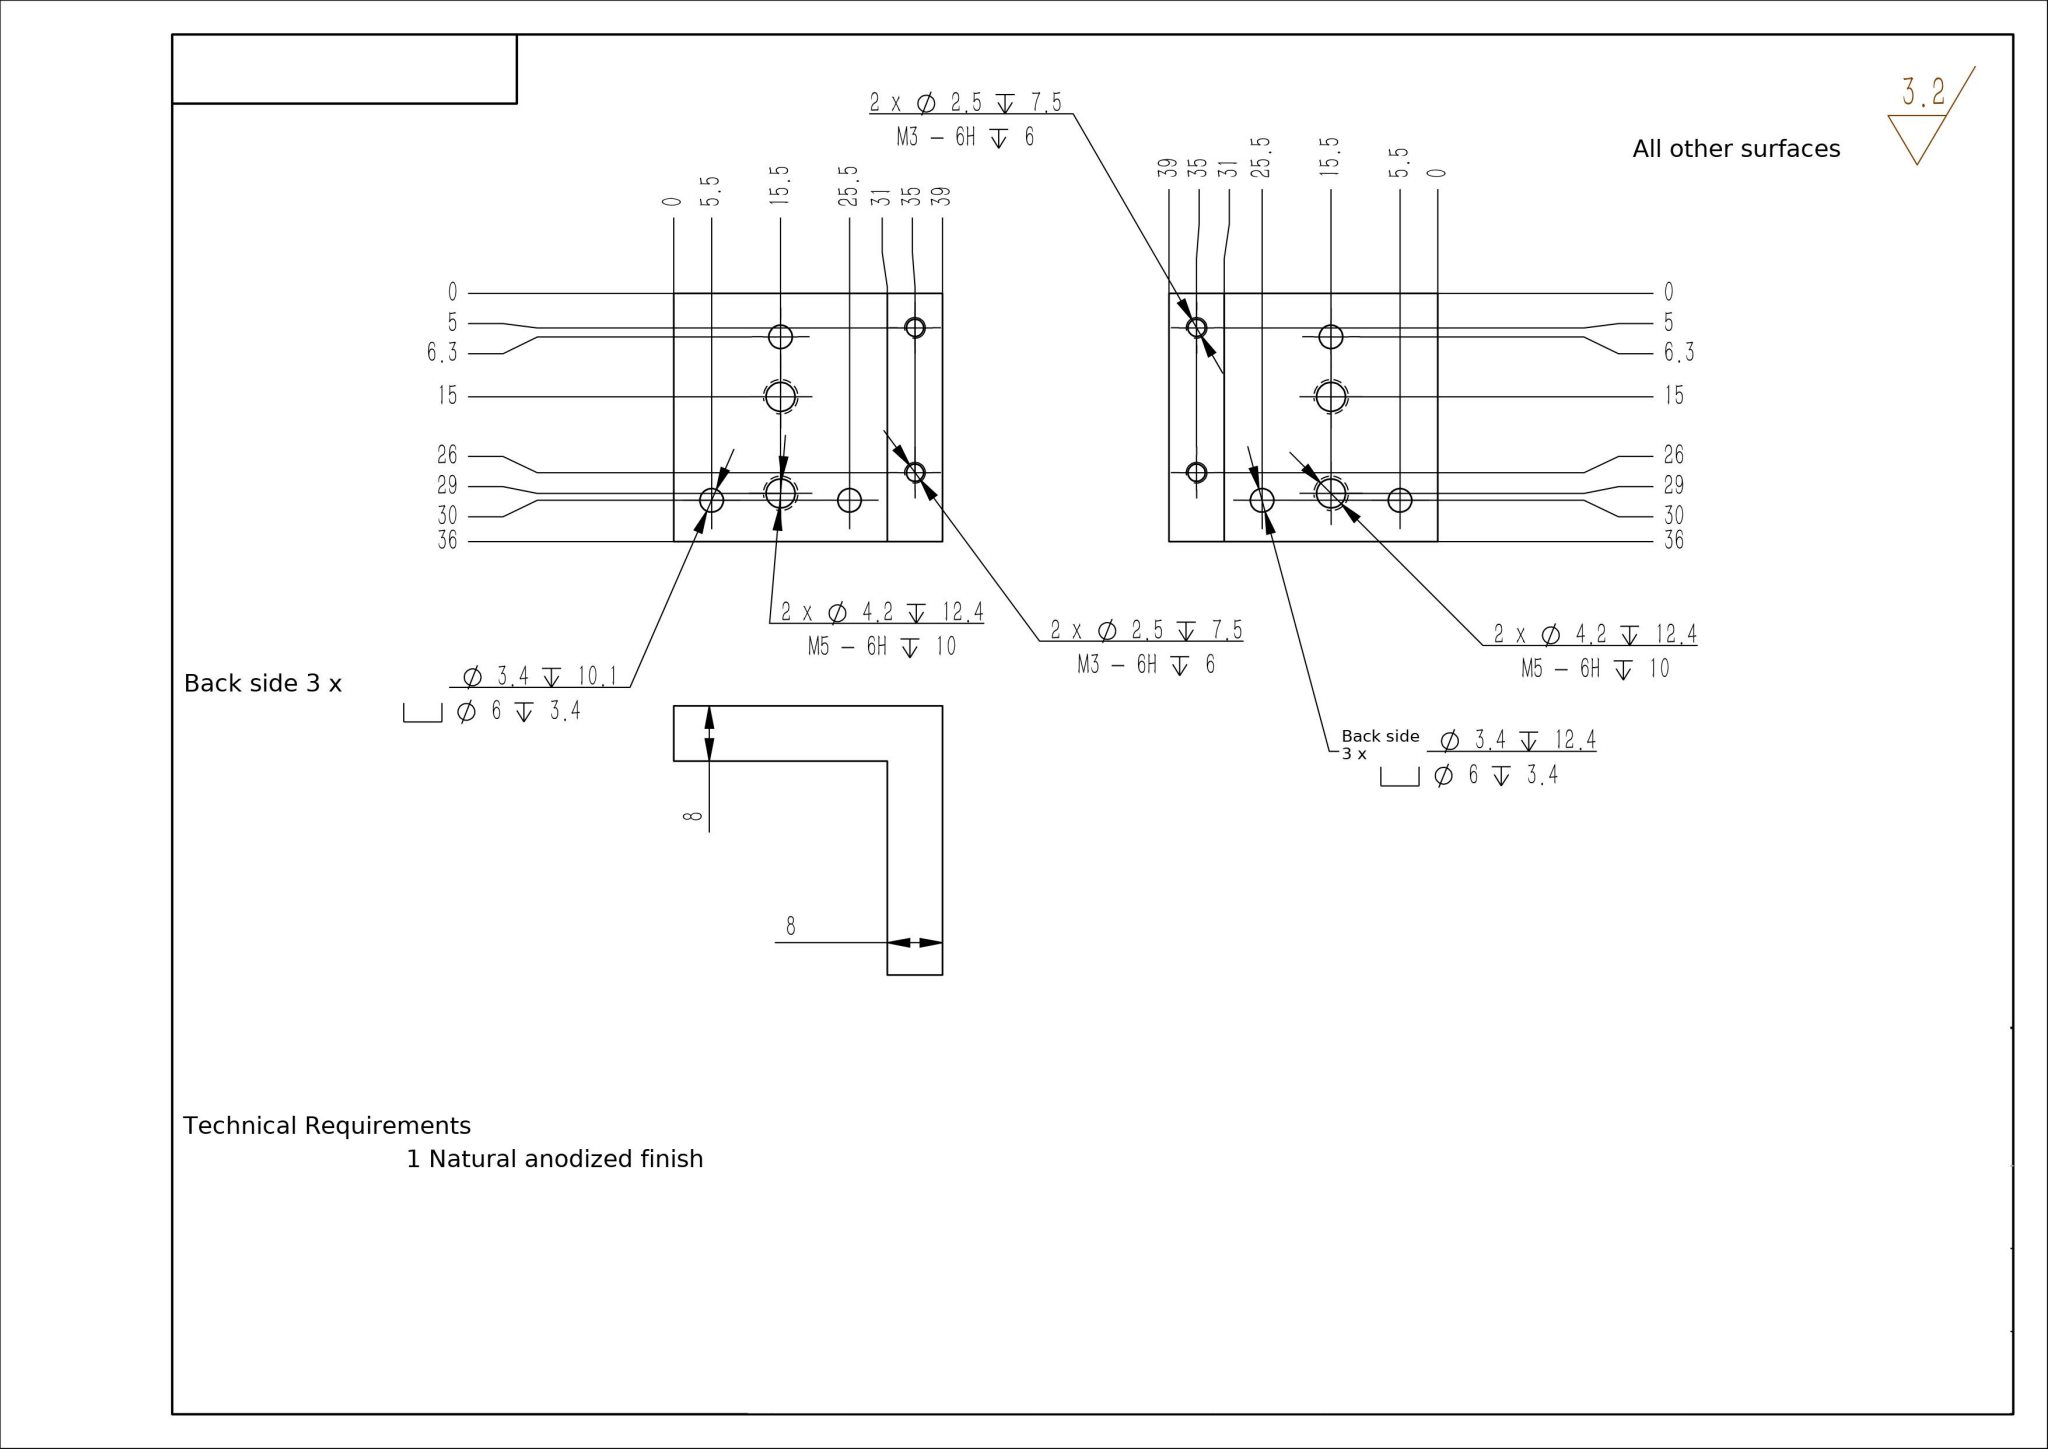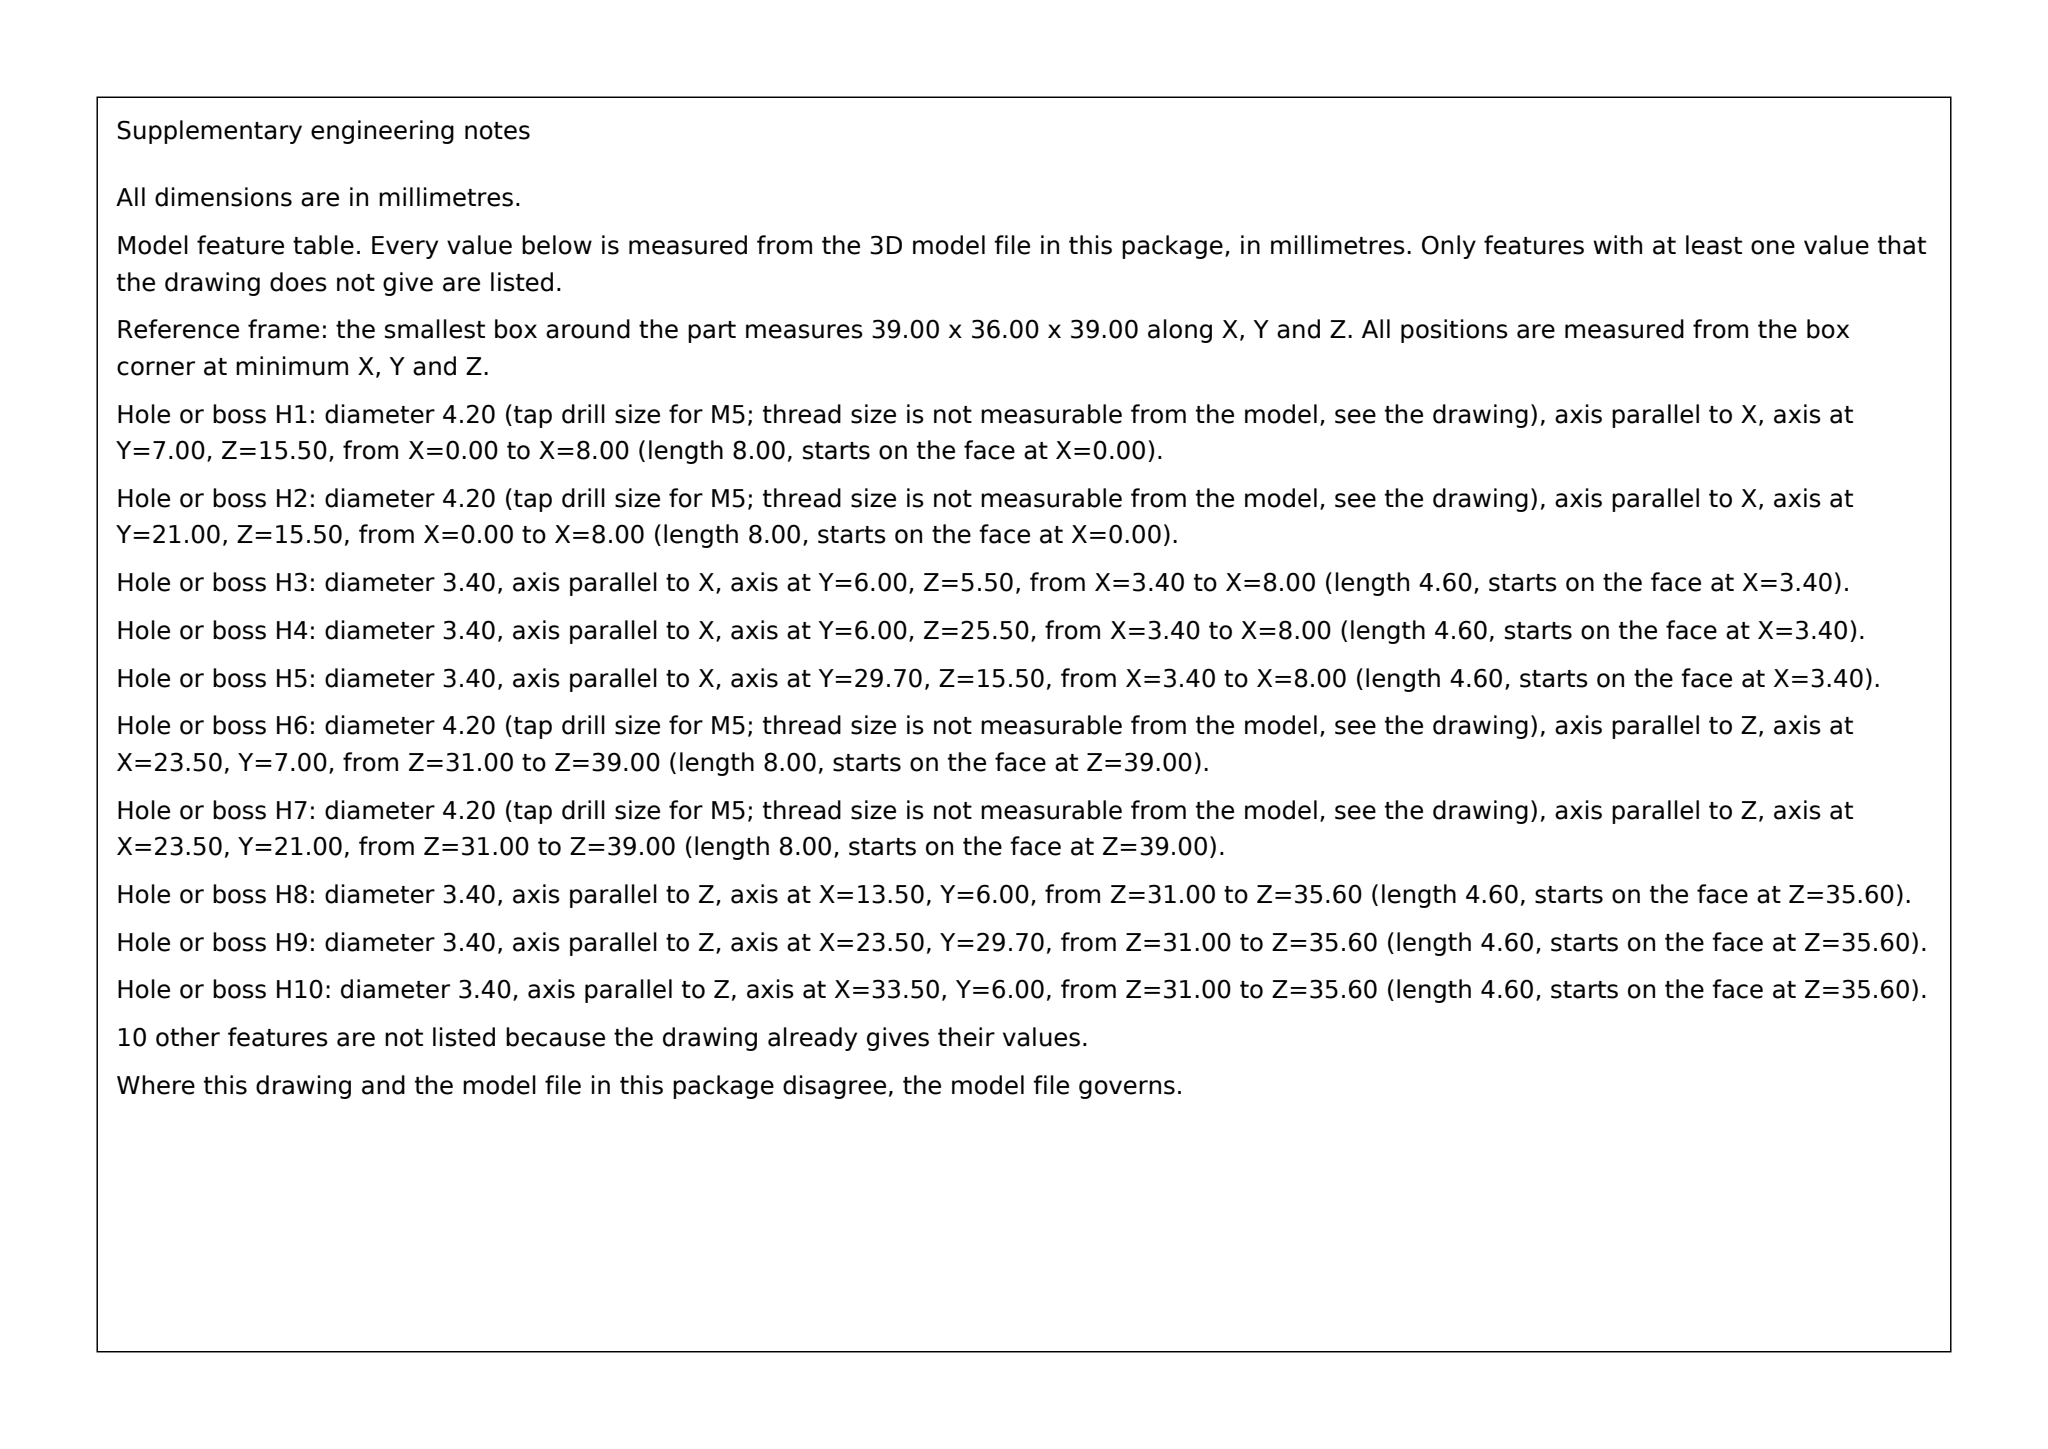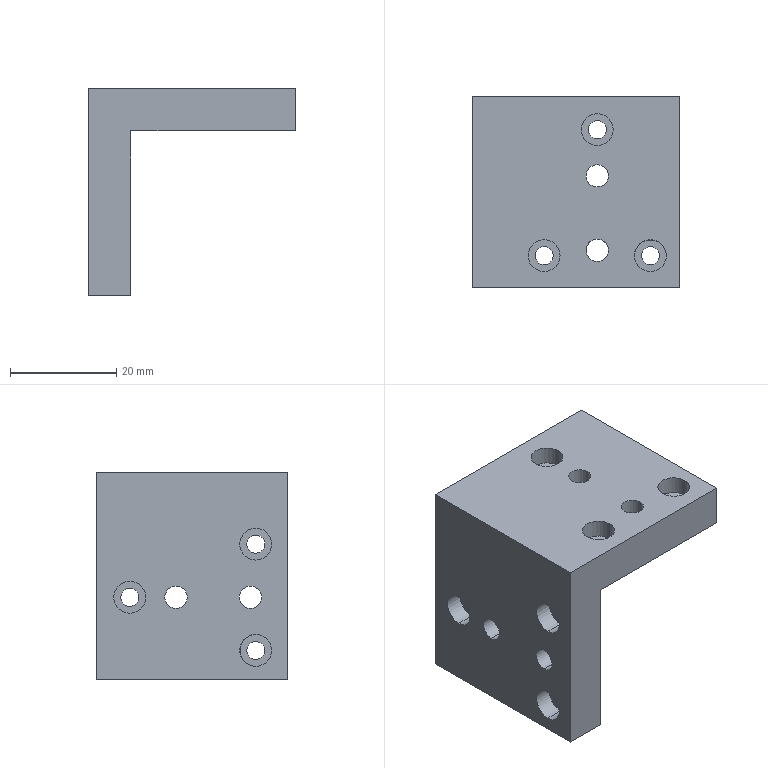Part | SolidWorks | mm | 1 solid | 62 faces | box 39 x 36 x 39 mm | volume 18737 mm3 | cylinder 40 | plane 14 | cone 8 | commonest cylinder face diameters 6 x12 3.4 x12 2.5 x8 4.2 x8
build123d program:
from build123d import *

# Parameters (mm, degrees)
BOSS_EXTRUDE1_DEPTH                               = 36
HOLE_SIZE_ACCORDING_TO_HEXAGON_SOCKET_D           = 3.4
HOLE_SIZE_ACCORDING_TO_HEXAGON_SOCKET_DEPTH       = 10.1
HOLE_SIZE_ACCORDING_TO_HEXAGON_SOCKET_CBORE_D     = 6
HOLE_SIZE_ACCORDING_TO_HEXAGON_SOCKET_CBORE_DEPTH = 3.4
HOLE_SIZE_ACCORDING_TO_HEXAGON_SOCKET_TIP         = 1.021
M5_TAPPED_HOLE1_D                                 = 4.2
M5_TAPPED_HOLE1_DEPTH                             = 12.4
M5_TAPPED_HOLE1_TIP                               = 1.262
HOLE_SIZE_ACCORDING_TO_HEXAGON_SO_2_D             = 3.4
HOLE_SIZE_ACCORDING_TO_HEXAGON_SO_2_DEPTH         = 12.4
HOLE_SIZE_ACCORDING_TO_HEXAGON_SO_2_CBORE_D       = 6
HOLE_SIZE_ACCORDING_TO_HEXAGON_SO_2_CBORE_DEPTH   = 3.4
HOLE_SIZE_ACCORDING_TO_HEXAGON_SO_2_TIP           = 1.021
M5_TAPPED_HOLE2_D                                 = 4.2
M5_TAPPED_HOLE2_DEPTH                             = 12.4
M5_TAPPED_HOLE2_TIP                               = 1.262
M3_TAPPED_HOLE1_D                                 = 2.5
M3_TAPPED_HOLE1_DEPTH                             = 7.5
M3_TAPPED_HOLE1_TIP                               = 0.7511
M3_TAPPED_HOLE2_D                                 = 2.5
M3_TAPPED_HOLE2_DEPTH                             = 7.5
M3_TAPPED_HOLE2_TIP                               = 0.7511


with BuildPart() as part:
    # Sketch1 → Boss-Extrude1 (new body)
    with BuildSketch(Plane(origin=(0, 0, 0), x_dir=(1, 0, 0), z_dir=(0, 1, 0))):
        Polygon((-16.522, 24.826), (-16.522, -14.174), (22.478, -14.174), (22.478, -6.174), (-8.522, -6.174), (-8.522, 24.826), align=None)
    extrude(amount=BOSS_EXTRUDE1_DEPTH)

    # Hole Size _ according to_ Hexagon Socket
    with Locations(Plane.XY.offset(14.174)):
        with Locations((6.978, 29.7), (-3.022, 6), (16.978, 6)):
            CounterBoreHole(HOLE_SIZE_ACCORDING_TO_HEXAGON_SOCKET_D / 2, HOLE_SIZE_ACCORDING_TO_HEXAGON_SOCKET_CBORE_D / 2, HOLE_SIZE_ACCORDING_TO_HEXAGON_SOCKET_CBORE_DEPTH, depth=HOLE_SIZE_ACCORDING_TO_HEXAGON_SOCKET_DEPTH)
            with Locations((0, 0, -(HOLE_SIZE_ACCORDING_TO_HEXAGON_SOCKET_DEPTH + HOLE_SIZE_ACCORDING_TO_HEXAGON_SOCKET_TIP / 2))):  # 118° drill point
                Cone(0, HOLE_SIZE_ACCORDING_TO_HEXAGON_SOCKET_D / 2, HOLE_SIZE_ACCORDING_TO_HEXAGON_SOCKET_TIP, mode=Mode.SUBTRACT)

    # M5 Tapped Hole1
    with Locations(Plane.XY.offset(14.174)):
        with Locations((6.977, 21), (6.977, 7)):
            Hole(M5_TAPPED_HOLE1_D / 2, depth=M5_TAPPED_HOLE1_DEPTH)
            with Locations((0, 0, -(M5_TAPPED_HOLE1_DEPTH + M5_TAPPED_HOLE1_TIP / 2))):  # 118° drill point
                Cone(0, M5_TAPPED_HOLE1_D / 2, M5_TAPPED_HOLE1_TIP, mode=Mode.SUBTRACT)

    # Hole Size _ according to_ Hexagon So 2
    with Locations(Plane.ZY.offset(16.522)):
        with Locations((-9.326, 29.7), (-19.326, 6), (0.6739, 6)):
            CounterBoreHole(HOLE_SIZE_ACCORDING_TO_HEXAGON_SO_2_D / 2, HOLE_SIZE_ACCORDING_TO_HEXAGON_SO_2_CBORE_D / 2, HOLE_SIZE_ACCORDING_TO_HEXAGON_SO_2_CBORE_DEPTH, depth=HOLE_SIZE_ACCORDING_TO_HEXAGON_SO_2_DEPTH)
            with Locations((0, 0, -(HOLE_SIZE_ACCORDING_TO_HEXAGON_SO_2_DEPTH + HOLE_SIZE_ACCORDING_TO_HEXAGON_SO_2_TIP / 2))):  # 118° drill point
                Cone(0, HOLE_SIZE_ACCORDING_TO_HEXAGON_SO_2_D / 2, HOLE_SIZE_ACCORDING_TO_HEXAGON_SO_2_TIP, mode=Mode.SUBTRACT)

    # M5 Tapped Hole2
    with Locations(Plane.ZY.offset(16.522)):
        with Locations((-9.326, 21), (-9.326, 7)):
            Hole(M5_TAPPED_HOLE2_D / 2, depth=M5_TAPPED_HOLE2_DEPTH)
            with Locations((0, 0, -(M5_TAPPED_HOLE2_DEPTH + M5_TAPPED_HOLE2_TIP / 2))):  # 118° drill point
                Cone(0, M5_TAPPED_HOLE2_D / 2, M5_TAPPED_HOLE2_TIP, mode=Mode.SUBTRACT)

    # M3 Tapped Hole1
    with Locations(Plane(origin=(0, 0, -24.826), x_dir=(-1, 0, 0), z_dir=(0, 0, -1))):
        with Locations((12.522, 31), (12.522, 10)):
            Hole(M3_TAPPED_HOLE1_D / 2, depth=M3_TAPPED_HOLE1_DEPTH)
            with Locations((0, 0, -(M3_TAPPED_HOLE1_DEPTH + M3_TAPPED_HOLE1_TIP / 2))):  # 118° drill point
                Cone(0, M3_TAPPED_HOLE1_D / 2, M3_TAPPED_HOLE1_TIP, mode=Mode.SUBTRACT)

    # M3 Tapped Hole2
    with Locations(Plane(origin=(22.478, 0, 0), x_dir=(0, 0, -1), z_dir=(1, 0, 0))):
        with Locations((-10.174, 31), (-10.174, 10)):
            Hole(M3_TAPPED_HOLE2_D / 2, depth=M3_TAPPED_HOLE2_DEPTH)
            with Locations((0, 0, -(M3_TAPPED_HOLE2_DEPTH + M3_TAPPED_HOLE2_TIP / 2))):  # 118° drill point
                Cone(0, M3_TAPPED_HOLE2_D / 2, M3_TAPPED_HOLE2_TIP, mode=Mode.SUBTRACT)


solid = part.part